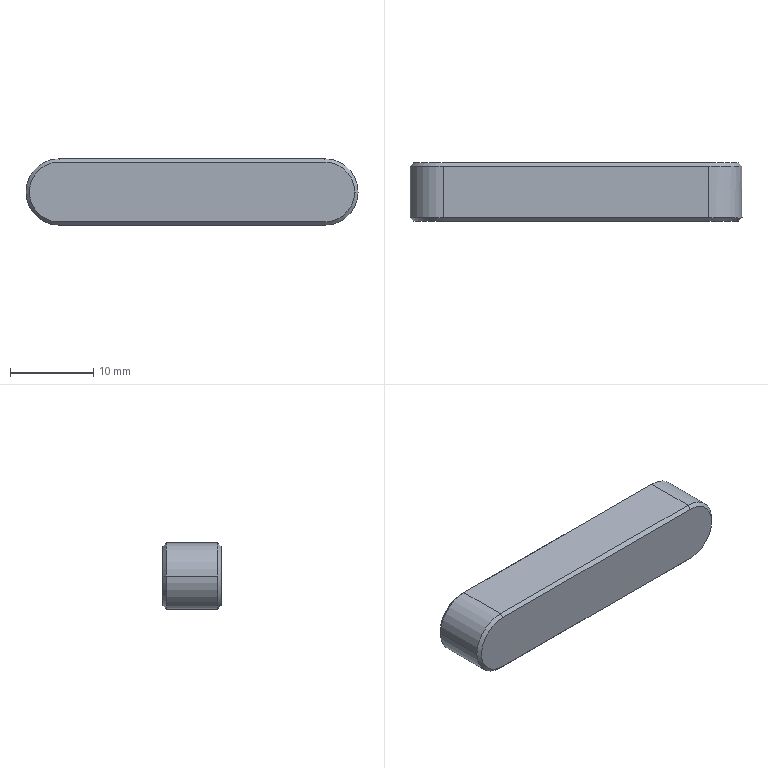Component | SolidWorks | Key8-7-40-1 | 1 solid | 17 faces | box 40 x 7 x 8 mm | volume 2130 mm3 | plane 8 | cone 6 | cylinder 3 | commonest cylinder face diameters 8 x3
build123d program:
from build123d import *

# Parameters (mm, degrees)
BOSS_EXTRUDE1_DEPTH = 7
CHAMFER1_SIZE2      = 0.4
CHAMFER1_SIZE       = 0.4


with BuildPart() as part:
    # Sketch1 → Boss-Extrude1 (new body)
    with BuildSketch(Plane(origin=(0, 0, 4), x_dir=(1, 0, 0), z_dir=(0, -1, 0))):
        with BuildLine():
            Line((-4, 28), (-4, -4))
            ThreePointArc((-4, -4), (0, -8), (4, -4))
            Line((4, -4), (4, 28))
            ThreePointArc((4, 28), (0, 32), (-4, 28))
        make_face()
    extrude(amount=-BOSS_EXTRUDE1_DEPTH)

    # Chamfer1
    chamfer1_edges = [part.edges().sort_by_distance(p)[0] for p in [
        (0, 7, -4),
        (4, 7, 16),
        (0, 7, 36),
        (4, 0, 16),
        (0, 0, -4),
        (-4, 0, 16),
        (0, 0, 36),
        (-4, 7, 16),
    ]]
    chamfer(chamfer1_edges, length=CHAMFER1_SIZE, length2=CHAMFER1_SIZE2)


solid = part.part

# Placed as in the assembly
solid = solid.moved(Location((-558.976, -122, 440.206), (0, 90, 0)))
STEP:
#1=COLOUR_RGB('',0.7922,0.8196,0.9333);
#2=FILL_AREA_STYLE_COLOUR('',#1);
#3=FILL_AREA_STYLE('',(#2));
#4=SURFACE_STYLE_FILL_AREA(#3);
#5=SURFACE_SIDE_STYLE('',(#4));
#6=SURFACE_STYLE_USAGE(.BOTH.,#5);
#7=PRESENTATION_STYLE_ASSIGNMENT((#6));
#8=CARTESIAN_POINT('',(-22.149,-4.528,17.331));
#9=VERTEX_POINT('',#8);
#10=CARTESIAN_POINT('',(-22.007,-4.528,17.473));
#11=VERTEX_POINT('',#10);
#12=CARTESIAN_POINT('',(-22.007,-4.528,17.331));
#13=DIRECTION('',(0.,1.,0.));
#14=DIRECTION('',(-1.,0.,0.));
#15=AXIS2_PLACEMENT_3D('',#12,#13,#14);
#16=CIRCLE('',#15,0.1417);
#17=EDGE_CURVE('',#9,#11,#16,.T.);
#18=ORIENTED_EDGE('',*,*,#17,.F.);
#19=CARTESIAN_POINT('',(-22.164,-4.543,17.331));
#20=VERTEX_POINT('',#19);
#21=CARTESIAN_POINT('',(-22.164,-4.543,17.331));
#22=DIRECTION('',(-0.7071,-0.7071,0.));
#23=VECTOR('',#22,39.37);
#24=LINE('',#21,#23);
#25=EDGE_CURVE('',#9,#20,#24,.T.);
#26=ORIENTED_EDGE('',*,*,#25,.T.);
#27=CARTESIAN_POINT('',(-22.007,-4.543,17.488));
#28=VERTEX_POINT('',#27);
#29=CARTESIAN_POINT('',(-22.007,-4.543,17.331));
#30=DIRECTION('',(0.,-1.,0.));
#31=DIRECTION('',(-1.,0.,0.));
#32=AXIS2_PLACEMENT_3D('',#29,#30,#31);
#33=CIRCLE('',#32,0.1575);
#34=EDGE_CURVE('',#28,#20,#33,.T.);
#35=ORIENTED_EDGE('',*,*,#34,.F.);
#36=CARTESIAN_POINT('',(-22.007,-4.528,17.473));
#37=DIRECTION('',(0.,-0.7071,0.7071));
#38=VECTOR('',#37,39.37);
#39=LINE('',#36,#38);
#40=EDGE_CURVE('',#11,#28,#39,.T.);
#41=ORIENTED_EDGE('',*,*,#40,.F.);
#42=EDGE_LOOP('',(#18,#26,#35,#41));
#43=FACE_OUTER_BOUND('',#42,.T.);
#44=CARTESIAN_POINT('',(-22.007,-4.543,17.331));
#45=DIRECTION('',(0.,-1.,0.));
#46=DIRECTION('',(-1.,0.,0.));
#47=AXIS2_PLACEMENT_3D('',#44,#45,#46);
#48=CONICAL_SURFACE('',#47,0.1575,0.7854);
#49=ADVANCED_FACE('',(#43),#48,.T.);
#50=CARTESIAN_POINT('',(-20.605,-4.803,17.331));
#51=VERTEX_POINT('',#50);
#52=CARTESIAN_POINT('',(-20.747,-4.803,17.473));
#53=VERTEX_POINT('',#52);
#54=CARTESIAN_POINT('',(-20.747,-4.803,17.331));
#55=DIRECTION('',(0.,-1.,0.));
#56=DIRECTION('',(-1.,0.,0.));
#57=AXIS2_PLACEMENT_3D('',#54,#55,#56);
#58=CIRCLE('',#57,0.1417);
#59=EDGE_CURVE('',#51,#53,#58,.T.);
#60=ORIENTED_EDGE('',*,*,#59,.F.);
#61=CARTESIAN_POINT('',(-20.59,-4.787,17.331));
#62=VERTEX_POINT('',#61);
#63=CARTESIAN_POINT('',(-20.605,-4.803,17.331));
#64=DIRECTION('',(0.7071,0.7071,-0.));
#65=VECTOR('',#64,39.37);
#66=LINE('',#63,#65);
#67=EDGE_CURVE('',#51,#62,#66,.T.);
#68=ORIENTED_EDGE('',*,*,#67,.T.);
#69=CARTESIAN_POINT('',(-20.747,-4.787,17.488));
#70=VERTEX_POINT('',#69);
#71=CARTESIAN_POINT('',(-20.747,-4.787,17.331));
#72=DIRECTION('',(0.,1.,0.));
#73=DIRECTION('',(-1.,0.,0.));
#74=AXIS2_PLACEMENT_3D('',#71,#72,#73);
#75=CIRCLE('',#74,0.1575);
#76=EDGE_CURVE('',#70,#62,#75,.T.);
#77=ORIENTED_EDGE('',*,*,#76,.F.);
#78=CARTESIAN_POINT('',(-20.747,-4.787,17.488));
#79=DIRECTION('',(-0.,-0.7071,-0.7071));
#80=VECTOR('',#79,39.37);
#81=LINE('',#78,#80);
#82=EDGE_CURVE('',#70,#53,#81,.T.);
#83=ORIENTED_EDGE('',*,*,#82,.T.);
#84=EDGE_LOOP('',(#60,#68,#77,#83));
#85=FACE_OUTER_BOUND('',#84,.T.);
#86=CARTESIAN_POINT('',(-20.747,-4.803,17.331));
#87=DIRECTION('',(0.,1.,0.));
#88=DIRECTION('',(1.,0.,0.));
#89=AXIS2_PLACEMENT_3D('',#86,#87,#88);
#90=CONICAL_SURFACE('',#89,0.1417,0.7854);
#91=ADVANCED_FACE('',(#85),#90,.T.);
#92=ORIENTED_EDGE('',*,*,#34,.T.);
#93=CARTESIAN_POINT('',(-22.164,-4.787,17.331));
#94=VERTEX_POINT('',#93);
#95=CARTESIAN_POINT('',(-22.164,-4.528,17.331));
#96=DIRECTION('',(0.,-1.,0.));
#97=VECTOR('',#96,39.37);
#98=LINE('',#95,#97);
#99=EDGE_CURVE('',#20,#94,#98,.T.);
#100=ORIENTED_EDGE('',*,*,#99,.T.);
#101=CARTESIAN_POINT('',(-22.007,-4.787,17.488));
#102=VERTEX_POINT('',#101);
#103=CARTESIAN_POINT('',(-22.007,-4.787,17.331));
#104=DIRECTION('',(0.,1.,0.));
#105=DIRECTION('',(-1.,0.,0.));
#106=AXIS2_PLACEMENT_3D('',#103,#104,#105);
#107=CIRCLE('',#106,0.1575);
#108=EDGE_CURVE('',#94,#102,#107,.T.);
#109=ORIENTED_EDGE('',*,*,#108,.T.);
#110=CARTESIAN_POINT('',(-22.007,-4.528,17.488));
#111=DIRECTION('',(0.,-1.,0.));
#112=VECTOR('',#111,39.37);
#113=LINE('',#110,#112);
#114=EDGE_CURVE('',#28,#102,#113,.T.);
#115=ORIENTED_EDGE('',*,*,#114,.F.);
#116=EDGE_LOOP('',(#92,#100,#109,#115));
#117=FACE_OUTER_BOUND('',#116,.T.);
#118=CARTESIAN_POINT('',(-22.007,-4.528,17.331));
#119=DIRECTION('',(0.,-1.,0.));
#120=DIRECTION('',(-1.,0.,0.));
#121=AXIS2_PLACEMENT_3D('',#118,#119,#120);
#122=CYLINDRICAL_SURFACE('',#121,0.1575);
#123=ADVANCED_FACE('',(#117),#122,.T.);
#124=CARTESIAN_POINT('',(-20.747,-4.543,17.488));
#125=VERTEX_POINT('',#124);
#126=CARTESIAN_POINT('',(-20.747,-4.528,17.488));
#127=DIRECTION('',(0.,-1.,0.));
#128=VECTOR('',#127,39.37);
#129=LINE('',#126,#128);
#130=EDGE_CURVE('',#125,#70,#129,.T.);
#131=ORIENTED_EDGE('',*,*,#130,.T.);
#132=ORIENTED_EDGE('',*,*,#76,.T.);
#133=CARTESIAN_POINT('',(-20.747,-4.787,17.173));
#134=VERTEX_POINT('',#133);
#135=CARTESIAN_POINT('',(-20.747,-4.787,17.331));
#136=DIRECTION('',(0.,1.,0.));
#137=DIRECTION('',(-1.,0.,0.));
#138=AXIS2_PLACEMENT_3D('',#135,#136,#137);
#139=CIRCLE('',#138,0.1575);
#140=EDGE_CURVE('',#62,#134,#139,.T.);
#141=ORIENTED_EDGE('',*,*,#140,.T.);
#142=CARTESIAN_POINT('',(-20.747,-4.543,17.173));
#143=VERTEX_POINT('',#142);
#144=CARTESIAN_POINT('',(-20.747,-4.528,17.173));
#145=DIRECTION('',(0.,-1.,0.));
#146=VECTOR('',#145,39.37);
#147=LINE('',#144,#146);
#148=EDGE_CURVE('',#143,#134,#147,.T.);
#149=ORIENTED_EDGE('',*,*,#148,.F.);
#150=CARTESIAN_POINT('',(-20.747,-4.543,17.331));
#151=DIRECTION('',(0.,-1.,0.));
#152=DIRECTION('',(-1.,0.,0.));
#153=AXIS2_PLACEMENT_3D('',#150,#151,#152);
#154=CIRCLE('',#153,0.1575);
#155=EDGE_CURVE('',#143,#125,#154,.T.);
#156=ORIENTED_EDGE('',*,*,#155,.T.);
#157=EDGE_LOOP('',(#131,#132,#141,#149,#156));
#158=FACE_OUTER_BOUND('',#157,.T.);
#159=CARTESIAN_POINT('',(-20.747,-4.528,17.331));
#160=DIRECTION('',(0.,-1.,0.));
#161=DIRECTION('',(-1.,0.,0.));
#162=AXIS2_PLACEMENT_3D('',#159,#160,#161);
#163=CYLINDRICAL_SURFACE('',#162,0.1575);
#164=ADVANCED_FACE('',(#158),#163,.T.);
#165=ORIENTED_EDGE('',*,*,#148,.T.);
#166=CARTESIAN_POINT('',(-22.007,-4.787,17.173));
#167=VERTEX_POINT('',#166);
#168=CARTESIAN_POINT('',(-22.007,-4.787,17.173));
#169=DIRECTION('',(-1.,0.,0.));
#170=VECTOR('',#169,39.37);
#171=LINE('',#168,#170);
#172=EDGE_CURVE('',#134,#167,#171,.T.);
#173=ORIENTED_EDGE('',*,*,#172,.T.);
#174=CARTESIAN_POINT('',(-22.007,-4.543,17.173));
#175=VERTEX_POINT('',#174);
#176=CARTESIAN_POINT('',(-22.007,-4.528,17.173));
#177=DIRECTION('',(0.,-1.,0.));
#178=VECTOR('',#177,39.37);
#179=LINE('',#176,#178);
#180=EDGE_CURVE('',#175,#167,#179,.T.);
#181=ORIENTED_EDGE('',*,*,#180,.F.);
#182=CARTESIAN_POINT('',(-20.747,-4.543,17.173));
#183=DIRECTION('',(1.,0.,-0.));
#184=VECTOR('',#183,39.37);
#185=LINE('',#182,#184);
#186=EDGE_CURVE('',#175,#143,#185,.T.);
#187=ORIENTED_EDGE('',*,*,#186,.T.);
#188=EDGE_LOOP('',(#165,#173,#181,#187));
#189=FACE_OUTER_BOUND('',#188,.T.);
#190=CARTESIAN_POINT('',(-22.007,-4.528,17.173));
#191=DIRECTION('',(-0.,0.,-1.));
#192=DIRECTION('',(-1.,0.,0.));
#193=AXIS2_PLACEMENT_3D('',#190,#191,#192);
#194=PLANE('',#193);
#195=ADVANCED_FACE('',(#189),#194,.T.);
#196=ORIENTED_EDGE('',*,*,#99,.F.);
#197=CARTESIAN_POINT('',(-22.007,-4.543,17.331));
#198=DIRECTION('',(0.,-1.,0.));
#199=DIRECTION('',(-1.,0.,0.));
#200=AXIS2_PLACEMENT_3D('',#197,#198,#199);
#201=CIRCLE('',#200,0.1575);
#202=EDGE_CURVE('',#20,#175,#201,.T.);
#203=ORIENTED_EDGE('',*,*,#202,.T.);
#204=ORIENTED_EDGE('',*,*,#180,.T.);
#205=CARTESIAN_POINT('',(-22.007,-4.787,17.331));
#206=DIRECTION('',(0.,1.,0.));
#207=DIRECTION('',(-1.,0.,0.));
#208=AXIS2_PLACEMENT_3D('',#205,#206,#207);
#209=CIRCLE('',#208,0.1575);
#210=EDGE_CURVE('',#167,#94,#209,.T.);
#211=ORIENTED_EDGE('',*,*,#210,.T.);
#212=EDGE_LOOP('',(#196,#203,#204,#211));
#213=FACE_OUTER_BOUND('',#212,.T.);
#214=CARTESIAN_POINT('',(-22.007,-4.528,17.331));
#215=DIRECTION('',(0.,-1.,0.));
#216=DIRECTION('',(-1.,0.,0.));
#217=AXIS2_PLACEMENT_3D('',#214,#215,#216);
#218=CYLINDRICAL_SURFACE('',#217,0.1575);
#219=ADVANCED_FACE('',(#213),#218,.T.);
#220=ORIENTED_EDGE('',*,*,#114,.T.);
#221=CARTESIAN_POINT('',(-20.747,-4.787,17.488));
#222=DIRECTION('',(1.,0.,-0.));
#223=VECTOR('',#222,39.37);
#224=LINE('',#221,#223);
#225=EDGE_CURVE('',#102,#70,#224,.T.);
#226=ORIENTED_EDGE('',*,*,#225,.T.);
#227=ORIENTED_EDGE('',*,*,#130,.F.);
#228=CARTESIAN_POINT('',(-22.007,-4.543,17.488));
#229=DIRECTION('',(-1.,0.,0.));
#230=VECTOR('',#229,39.37);
#231=LINE('',#228,#230);
#232=EDGE_CURVE('',#125,#28,#231,.T.);
#233=ORIENTED_EDGE('',*,*,#232,.T.);
#234=EDGE_LOOP('',(#220,#226,#227,#233));
#235=FACE_OUTER_BOUND('',#234,.T.);
#236=CARTESIAN_POINT('',(-20.747,-4.528,17.488));
#237=DIRECTION('',(0.,0.,1.));
#238=DIRECTION('',(1.,0.,-0.));
#239=AXIS2_PLACEMENT_3D('',#236,#237,#238);
#240=PLANE('',#239);
#241=ADVANCED_FACE('',(#235),#240,.T.);
#242=CARTESIAN_POINT('',(-22.007,-4.528,17.189));
#243=VERTEX_POINT('',#242);
#244=CARTESIAN_POINT('',(-22.007,-4.528,17.331));
#245=DIRECTION('',(0.,1.,0.));
#246=DIRECTION('',(-1.,0.,0.));
#247=AXIS2_PLACEMENT_3D('',#244,#245,#246);
#248=CIRCLE('',#247,0.1417);
#249=EDGE_CURVE('',#243,#9,#248,.T.);
#250=ORIENTED_EDGE('',*,*,#249,.T.);
#251=ORIENTED_EDGE('',*,*,#17,.T.);
#252=CARTESIAN_POINT('',(-20.747,-4.528,17.473));
#253=VERTEX_POINT('',#252);
#254=CARTESIAN_POINT('',(-20.747,-4.528,17.473));
#255=DIRECTION('',(1.,0.,-0.));
#256=VECTOR('',#255,39.37);
#257=LINE('',#254,#256);
#258=EDGE_CURVE('',#11,#253,#257,.T.);
#259=ORIENTED_EDGE('',*,*,#258,.T.);
#260=CARTESIAN_POINT('',(-20.747,-4.528,17.189));
#261=VERTEX_POINT('',#260);
#262=CARTESIAN_POINT('',(-20.747,-4.528,17.331));
#263=DIRECTION('',(0.,1.,0.));
#264=DIRECTION('',(-1.,0.,0.));
#265=AXIS2_PLACEMENT_3D('',#262,#263,#264);
#266=CIRCLE('',#265,0.1417);
#267=EDGE_CURVE('',#253,#261,#266,.T.);
#268=ORIENTED_EDGE('',*,*,#267,.T.);
#269=CARTESIAN_POINT('',(-22.007,-4.528,17.189));
#270=DIRECTION('',(-1.,0.,0.));
#271=VECTOR('',#270,39.37);
#272=LINE('',#269,#271);
#273=EDGE_CURVE('',#261,#243,#272,.T.);
#274=ORIENTED_EDGE('',*,*,#273,.T.);
#275=EDGE_LOOP('',(#250,#251,#259,#268,#274));
#276=FACE_OUTER_BOUND('',#275,.T.);
#277=CARTESIAN_POINT('',(-20.747,-4.528,17.331));
#278=DIRECTION('',(0.,-1.,0.));
#279=DIRECTION('',(-1.,0.,0.));
#280=AXIS2_PLACEMENT_3D('',#277,#278,#279);
#281=PLANE('',#280);
#282=ADVANCED_FACE('',(#276),#281,.F.);
#283=CARTESIAN_POINT('',(-22.007,-4.803,17.473));
#284=VERTEX_POINT('',#283);
#285=CARTESIAN_POINT('',(-22.007,-4.803,17.189));
#286=VERTEX_POINT('',#285);
#287=CARTESIAN_POINT('',(-22.007,-4.803,17.331));
#288=DIRECTION('',(0.,-1.,0.));
#289=DIRECTION('',(-1.,0.,0.));
#290=AXIS2_PLACEMENT_3D('',#287,#288,#289);
#291=CIRCLE('',#290,0.1417);
#292=EDGE_CURVE('',#284,#286,#291,.T.);
#293=ORIENTED_EDGE('',*,*,#292,.T.);
#294=CARTESIAN_POINT('',(-20.747,-4.803,17.189));
#295=VERTEX_POINT('',#294);
#296=CARTESIAN_POINT('',(-20.747,-4.803,17.189));
#297=DIRECTION('',(1.,0.,-0.));
#298=VECTOR('',#297,39.37);
#299=LINE('',#296,#298);
#300=EDGE_CURVE('',#286,#295,#299,.T.);
#301=ORIENTED_EDGE('',*,*,#300,.T.);
#302=CARTESIAN_POINT('',(-20.747,-4.803,17.331));
#303=DIRECTION('',(0.,-1.,0.));
#304=DIRECTION('',(-1.,0.,0.));
#305=AXIS2_PLACEMENT_3D('',#302,#303,#304);
#306=CIRCLE('',#305,0.1417);
#307=EDGE_CURVE('',#295,#51,#306,.T.);
#308=ORIENTED_EDGE('',*,*,#307,.T.);
#309=ORIENTED_EDGE('',*,*,#59,.T.);
#310=CARTESIAN_POINT('',(-20.747,-4.803,17.473));
#311=DIRECTION('',(-1.,0.,0.));
#312=VECTOR('',#311,39.37);
#313=LINE('',#310,#312);
#314=EDGE_CURVE('',#53,#284,#313,.T.);
#315=ORIENTED_EDGE('',*,*,#314,.T.);
#316=EDGE_LOOP('',(#293,#301,#308,#309,#315));
#317=FACE_OUTER_BOUND('',#316,.T.);
#318=CARTESIAN_POINT('',(-20.747,-4.803,17.331));
#319=DIRECTION('',(0.,-1.,0.));
#320=DIRECTION('',(-1.,0.,0.));
#321=AXIS2_PLACEMENT_3D('',#318,#319,#320);
#322=PLANE('',#321);
#323=ADVANCED_FACE('',(#317),#322,.T.);
#324=ORIENTED_EDGE('',*,*,#82,.F.);
#325=ORIENTED_EDGE('',*,*,#225,.F.);
#326=CARTESIAN_POINT('',(-22.007,-4.803,17.473));
#327=DIRECTION('',(0.,0.7071,0.7071));
#328=VECTOR('',#327,39.37);
#329=LINE('',#326,#328);
#330=EDGE_CURVE('',#284,#102,#329,.T.);
#331=ORIENTED_EDGE('',*,*,#330,.F.);
#332=ORIENTED_EDGE('',*,*,#314,.F.);
#333=EDGE_LOOP('',(#324,#325,#331,#332));
#334=FACE_OUTER_BOUND('',#333,.T.);
#335=CARTESIAN_POINT('',(-20.747,-4.803,17.473));
#336=DIRECTION('',(-0.,0.7071,-0.7071));
#337=DIRECTION('',(-1.,0.,0.));
#338=AXIS2_PLACEMENT_3D('',#335,#336,#337);
#339=PLANE('',#338);
#340=ADVANCED_FACE('',(#334),#339,.F.);
#341=ORIENTED_EDGE('',*,*,#330,.T.);
#342=ORIENTED_EDGE('',*,*,#108,.F.);
#343=ORIENTED_EDGE('',*,*,#210,.F.);
#344=CARTESIAN_POINT('',(-22.007,-4.803,17.189));
#345=DIRECTION('',(-0.,0.7071,-0.7071));
#346=VECTOR('',#345,39.37);
#347=LINE('',#344,#346);
#348=EDGE_CURVE('',#286,#167,#347,.T.);
#349=ORIENTED_EDGE('',*,*,#348,.F.);
#350=ORIENTED_EDGE('',*,*,#292,.F.);
#351=EDGE_LOOP('',(#341,#342,#343,#349,#350));
#352=FACE_OUTER_BOUND('',#351,.T.);
#353=CARTESIAN_POINT('',(-22.007,-4.803,17.331));
#354=DIRECTION('',(0.,1.,0.));
#355=DIRECTION('',(1.,0.,0.));
#356=AXIS2_PLACEMENT_3D('',#353,#354,#355);
#357=CONICAL_SURFACE('',#356,0.1417,0.7854);
#358=ADVANCED_FACE('',(#352),#357,.T.);
#359=ORIENTED_EDGE('',*,*,#67,.F.);
#360=ORIENTED_EDGE('',*,*,#307,.F.);
#361=CARTESIAN_POINT('',(-20.747,-4.787,17.173));
#362=DIRECTION('',(0.,-0.7071,0.7071));
#363=VECTOR('',#362,39.37);
#364=LINE('',#361,#363);
#365=EDGE_CURVE('',#134,#295,#364,.T.);
#366=ORIENTED_EDGE('',*,*,#365,.F.);
#367=ORIENTED_EDGE('',*,*,#140,.F.);
#368=EDGE_LOOP('',(#359,#360,#366,#367));
#369=FACE_OUTER_BOUND('',#368,.T.);
#370=CARTESIAN_POINT('',(-20.747,-4.803,17.331));
#371=DIRECTION('',(0.,1.,0.));
#372=DIRECTION('',(1.,0.,0.));
#373=AXIS2_PLACEMENT_3D('',#370,#371,#372);
#374=CONICAL_SURFACE('',#373,0.1417,0.7854);
#375=ADVANCED_FACE('',(#369),#374,.T.);
#376=ORIENTED_EDGE('',*,*,#348,.T.);
#377=ORIENTED_EDGE('',*,*,#172,.F.);
#378=ORIENTED_EDGE('',*,*,#365,.T.);
#379=ORIENTED_EDGE('',*,*,#300,.F.);
#380=EDGE_LOOP('',(#376,#377,#378,#379));
#381=FACE_OUTER_BOUND('',#380,.T.);
#382=CARTESIAN_POINT('',(-20.747,-4.803,17.189));
#383=DIRECTION('',(0.,0.7071,0.7071));
#384=DIRECTION('',(1.,0.,-0.));
#385=AXIS2_PLACEMENT_3D('',#382,#383,#384);
#386=PLANE('',#385);
#387=ADVANCED_FACE('',(#381),#386,.F.);
#388=CARTESIAN_POINT('',(-22.007,-4.528,17.189));
#389=DIRECTION('',(-0.,-0.7071,-0.7071));
#390=VECTOR('',#389,39.37);
#391=LINE('',#388,#390);
#392=EDGE_CURVE('',#243,#175,#391,.T.);
#393=ORIENTED_EDGE('',*,*,#392,.F.);
#394=ORIENTED_EDGE('',*,*,#273,.F.);
#395=CARTESIAN_POINT('',(-20.747,-4.543,17.173));
#396=DIRECTION('',(0.,0.7071,0.7071));
#397=VECTOR('',#396,39.37);
#398=LINE('',#395,#397);
#399=EDGE_CURVE('',#143,#261,#398,.T.);
#400=ORIENTED_EDGE('',*,*,#399,.F.);
#401=ORIENTED_EDGE('',*,*,#186,.F.);
#402=EDGE_LOOP('',(#393,#394,#400,#401));
#403=FACE_OUTER_BOUND('',#402,.T.);
#404=CARTESIAN_POINT('',(-22.007,-4.543,17.173));
#405=DIRECTION('',(-0.,0.7071,-0.7071));
#406=DIRECTION('',(-1.,0.,0.));
#407=AXIS2_PLACEMENT_3D('',#404,#405,#406);
#408=PLANE('',#407);
#409=ADVANCED_FACE('',(#403),#408,.T.);
#410=ORIENTED_EDGE('',*,*,#399,.T.);
#411=ORIENTED_EDGE('',*,*,#267,.F.);
#412=CARTESIAN_POINT('',(-20.747,-4.543,17.488));
#413=DIRECTION('',(-0.,0.7071,-0.7071));
#414=VECTOR('',#413,39.37);
#415=LINE('',#412,#414);
#416=EDGE_CURVE('',#125,#253,#415,.T.);
#417=ORIENTED_EDGE('',*,*,#416,.F.);
#418=ORIENTED_EDGE('',*,*,#155,.F.);
#419=EDGE_LOOP('',(#410,#411,#417,#418));
#420=FACE_OUTER_BOUND('',#419,.T.);
#421=CARTESIAN_POINT('',(-20.747,-4.543,17.331));
#422=DIRECTION('',(0.,-1.,0.));
#423=DIRECTION('',(-1.,0.,0.));
#424=AXIS2_PLACEMENT_3D('',#421,#422,#423);
#425=CONICAL_SURFACE('',#424,0.1575,0.7854);
#426=ADVANCED_FACE('',(#420),#425,.T.);
#427=ORIENTED_EDGE('',*,*,#25,.F.);
#428=ORIENTED_EDGE('',*,*,#249,.F.);
#429=ORIENTED_EDGE('',*,*,#392,.T.);
#430=ORIENTED_EDGE('',*,*,#202,.F.);
#431=EDGE_LOOP('',(#427,#428,#429,#430));
#432=FACE_OUTER_BOUND('',#431,.T.);
#433=CARTESIAN_POINT('',(-22.007,-4.543,17.331));
#434=DIRECTION('',(0.,-1.,0.));
#435=DIRECTION('',(-1.,0.,0.));
#436=AXIS2_PLACEMENT_3D('',#433,#434,#435);
#437=CONICAL_SURFACE('',#436,0.1575,0.7854);
#438=ADVANCED_FACE('',(#432),#437,.T.);
#439=ORIENTED_EDGE('',*,*,#416,.T.);
#440=ORIENTED_EDGE('',*,*,#258,.F.);
#441=ORIENTED_EDGE('',*,*,#40,.T.);
#442=ORIENTED_EDGE('',*,*,#232,.F.);
#443=EDGE_LOOP('',(#439,#440,#441,#442));
#444=FACE_OUTER_BOUND('',#443,.T.);
#445=CARTESIAN_POINT('',(-20.747,-4.543,17.488));
#446=DIRECTION('',(0.,0.7071,0.7071));
#447=DIRECTION('',(1.,0.,-0.));
#448=AXIS2_PLACEMENT_3D('',#445,#446,#447);
#449=PLANE('',#448);
#450=ADVANCED_FACE('',(#444),#449,.T.);
#451=CLOSED_SHELL('',(#49,#91,#123,#164,#195,#219,#241,#282,#323,#340,#358,#375,#387,#409,#426,#438,#450));
#452=MANIFOLD_SOLID_BREP('',#451);
#453=STYLED_ITEM('',(#7),#452);
#454=PRESENTATION_LAYER_ASSIGNMENT('','',(#453));
#455=(LENGTH_UNIT()NAMED_UNIT(*)SI_UNIT($,.METRE.));
#456=LENGTH_MEASURE_WITH_UNIT(LENGTH_MEASURE(0.0254),#455);
#457=DIMENSIONAL_EXPONENTS(1.,0.,0.,0.,0.,0.,0.);
#458=(CONVERSION_BASED_UNIT('',#456)LENGTH_UNIT()NAMED_UNIT(#457));
#459=UNCERTAINTY_MEASURE_WITH_UNIT(LENGTH_MEASURE(0.00001),#458,'','');
#460=(NAMED_UNIT(*)PLANE_ANGLE_UNIT()SI_UNIT($,.RADIAN.));
#461=(NAMED_UNIT(*)SI_UNIT($,.STERADIAN.)SOLID_ANGLE_UNIT());
#462=(GEOMETRIC_REPRESENTATION_CONTEXT(3)GLOBAL_UNCERTAINTY_ASSIGNED_CONTEXT((#459))GLOBAL_UNIT_ASSIGNED_CONTEXT((#458,#460,#461))REPRESENTATION_CONTEXT('',''));
#463=MECHANICAL_DESIGN_GEOMETRIC_PRESENTATION_REPRESENTATION('',(#453),#462);
#464=CARTESIAN_POINT('',(0.,0.,0.));
#465=DIRECTION('',(0.,0.,1.));
#466=DIRECTION('',(1.,0.,0.));
#467=AXIS2_PLACEMENT_3D('',#464,#465,#466);
#468=(LENGTH_UNIT()NAMED_UNIT(*)SI_UNIT($,.METRE.));
#469=LENGTH_MEASURE_WITH_UNIT(LENGTH_MEASURE(0.0254),#468);
#470=DIMENSIONAL_EXPONENTS(1.,0.,0.,0.,0.,0.,0.);
#471=(CONVERSION_BASED_UNIT('',#469)LENGTH_UNIT()NAMED_UNIT(#470));
#472=UNCERTAINTY_MEASURE_WITH_UNIT(LENGTH_MEASURE(0.00001),#471,'','');
#473=(NAMED_UNIT(*)PLANE_ANGLE_UNIT()SI_UNIT($,.RADIAN.));
#474=(NAMED_UNIT(*)SI_UNIT($,.STERADIAN.)SOLID_ANGLE_UNIT());
#475=(GEOMETRIC_REPRESENTATION_CONTEXT(3)GLOBAL_UNCERTAINTY_ASSIGNED_CONTEXT((#472))GLOBAL_UNIT_ASSIGNED_CONTEXT((#471,#473,#474))REPRESENTATION_CONTEXT('',''));
#476=ADVANCED_BREP_SHAPE_REPRESENTATION('',(#452,#467),#475);